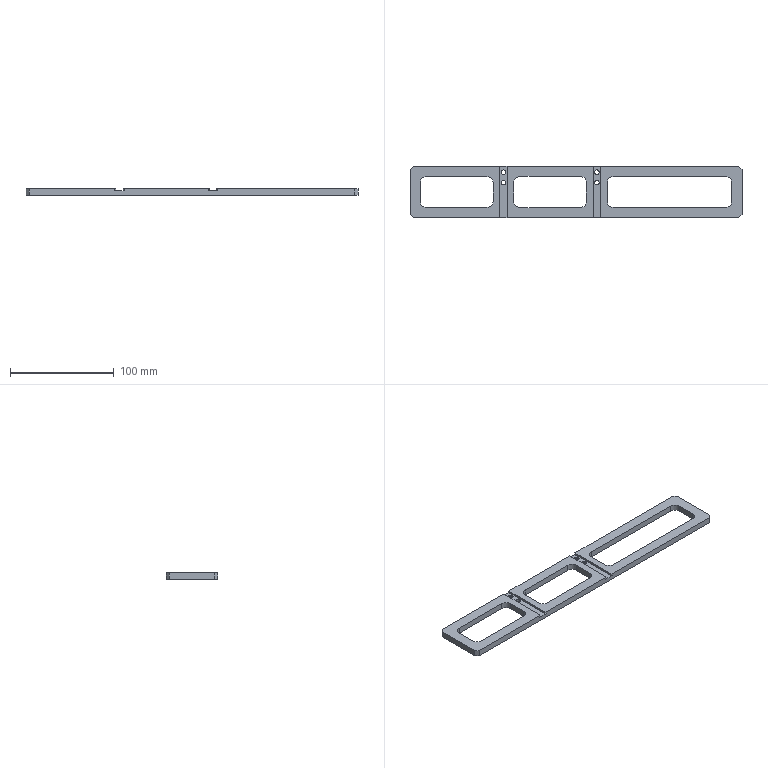Component | SolidWorks | OPW-05-008-1 | 1 solid | 62 faces | box 320 x 50 x 6 mm | volume 47781 mm3 | plane 34 | cylinder 20 | cone 8 | commonest cylinder face diameters 12 x12 4.5 x8
build123d program:
from build123d import *

# Parameters (mm, degrees)
SKETCH1_W                                            = 320
SKETCH1_H                                            = 50
BOSS_EXTRUDE1_DEPTH                                  = 3
COUNTERSUNK_HOLE_FOR_M4_HEX_SOCKET_COUNT_D           = 4.5
COUNTERSUNK_HOLE_FOR_M4_HEX_SOCKET_COUNT_CSINK_D     = 9.18
COUNTERSUNK_HOLE_FOR_M4_HEX_SOCKET_COUNT_CSINK_ANGLE = 90
SKETCH4_W                                            = 7
SKETCH4_H                                            = 50
CUT_EXTRUDE1_DEPTH                                   = 2
CHAMFER1_SIZE                                        = 1
CUT_EXTRUDE2_REACH                                   = 164.052
SKETCH5_W                                            = 70
SKETCH5_H                                            = 30
SKETCH5_W_2                                          = 120
FILLET1_R                                            = 6
CHAMFER2_SIZE                                        = 3


with BuildPart() as part:
    # Sketch1 → Boss-Extrude1 (new, symmetric)
    with BuildSketch(Plane.XY):
        Rectangle(SKETCH1_W, SKETCH1_H)
    extrude(amount=BOSS_EXTRUDE1_DEPTH, both=True)

    # Countersunk Hole for M4 Hex Socket Count (through all)
    with Locations(Plane(origin=(0, 0, -3), x_dir=(-1, 0, 0), z_dir=(0, 0, -1))):
        with Locations((70, 9), (-20, 9), (-20, 19), (70, 19)):
            CounterSinkHole(COUNTERSUNK_HOLE_FOR_M4_HEX_SOCKET_COUNT_D / 2, COUNTERSUNK_HOLE_FOR_M4_HEX_SOCKET_COUNT_CSINK_D / 2, counter_sink_angle=COUNTERSUNK_HOLE_FOR_M4_HEX_SOCKET_COUNT_CSINK_ANGLE)

    # Sketch4 → Cut-Extrude1 (cut)
    with BuildSketch(Plane.XY.offset(3)):
        with Locations((-70, 0)):
            Rectangle(SKETCH4_W, SKETCH4_H)
        with Locations((20, 0)):
            Rectangle(SKETCH4_W, SKETCH4_H)
    extrude(amount=-CUT_EXTRUDE1_DEPTH, mode=Mode.SUBTRACT)

    # Chamfer1
    chamfer1_edges = [part.edges().sort_by_distance(p)[0] for p in [
        (-73.5, -25, 2),
        (-66.5, -25, 2),
        (16.5, -25, 2),
        (23.5, -25, 2),
    ]]
    chamfer(chamfer1_edges, length=CHAMFER1_SIZE)

    # Sketch5 → Cut-Extrude2 (cut, up to next)
    with BuildSketch(Plane(origin=(0, 0, -3), x_dir=(-1, 0, 0), z_dir=(0, 0, -1)), mode=Mode.PRIVATE) as cut_extrude2_sk1:
        with Locations((115, 0)):
            Rectangle(SKETCH5_W, SKETCH5_H)
    cut_extrude2_tool1 = extrude(cut_extrude2_sk1.sketch, amount=-CUT_EXTRUDE2_REACH, mode=Mode.PRIVATE) & part.part
    # Sketch5 → Cut-Extrude2 (cut, up to next)
    with BuildSketch(Plane(origin=(0, 0, -3), x_dir=(-1, 0, 0), z_dir=(0, 0, -1)), mode=Mode.PRIVATE) as cut_extrude2_sk2:
        with Locations((25, 0)):
            Rectangle(SKETCH5_W, SKETCH5_H)
    cut_extrude2_tool2 = extrude(cut_extrude2_sk2.sketch, amount=-CUT_EXTRUDE2_REACH, mode=Mode.PRIVATE) & part.part
    # Sketch5 → Cut-Extrude2 (cut, up to next)
    with BuildSketch(Plane(origin=(0, 0, -3), x_dir=(-1, 0, 0), z_dir=(0, 0, -1)), mode=Mode.PRIVATE) as cut_extrude2_sk3:
        with Locations((-90, 0)):
            Rectangle(SKETCH5_W_2, SKETCH5_H)
    cut_extrude2_tool3 = extrude(cut_extrude2_sk3.sketch, amount=-CUT_EXTRUDE2_REACH, mode=Mode.PRIVATE) & part.part
    add(cut_extrude2_tool1.solids().sort_by_distance((-115, 0, -3))[0], mode=Mode.SUBTRACT)
    add(cut_extrude2_tool2.solids().sort_by_distance((-25, 0, -3))[0], mode=Mode.SUBTRACT)
    add(cut_extrude2_tool3.solids().sort_by_distance((90, 0, -3))[0], mode=Mode.SUBTRACT)

    # Fillet1
    fillet1_edges = [part.edges().sort_by_distance(p)[0] for p in [
        (-80, -15, 0),
        (-80, 15, 0),
        (-150, 15, 0),
        (-150, -15, 0),
        (10, -15, 0),
        (10, 15, 0),
        (-60, 15, 0),
        (-60, -15, 0),
        (150, -15, 0),
        (150, 15, 0),
        (30, 15, 0),
        (30, -15, 0),
    ]]
    fillet(fillet1_edges, radius=FILLET1_R)

    # Chamfer2
    chamfer2_edges = [part.edges().sort_by_distance(p)[0] for p in [
        (-160, 25, 0),
        (160, 25, 0),
        (160, -25, 0),
        (-160, -25, 0),
    ]]
    chamfer(chamfer2_edges, length=CHAMFER2_SIZE)


solid = part.part

# Placed as in the assembly
solid = solid.moved(Location((-79.904, 257.499, -46), (0, 0, 0)))